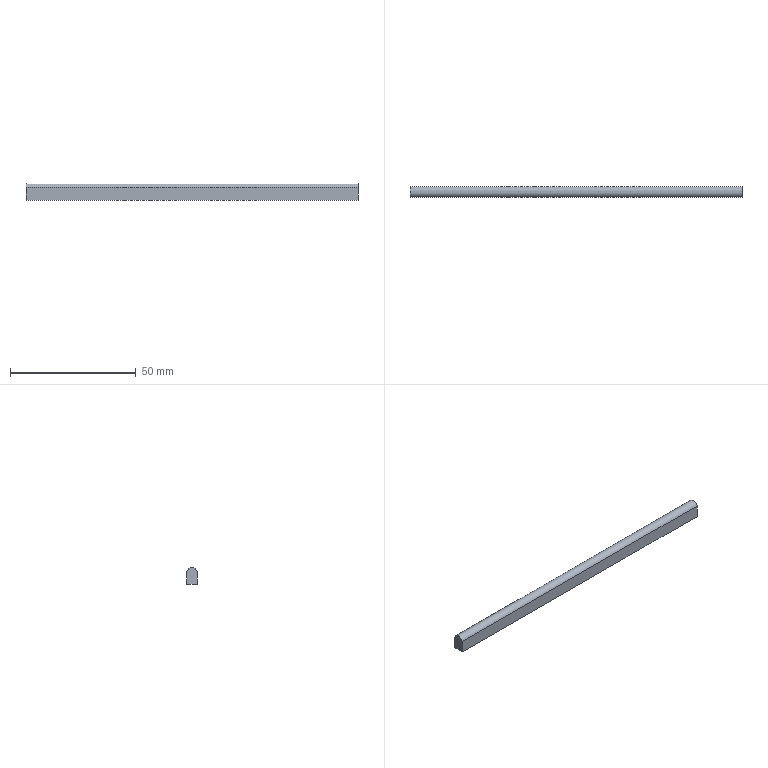CAM job | Mastercam | mm | 10 operations | part box 131.92 x 4.2 x 6.7
1. Facing | 10 - 10 平铣刀
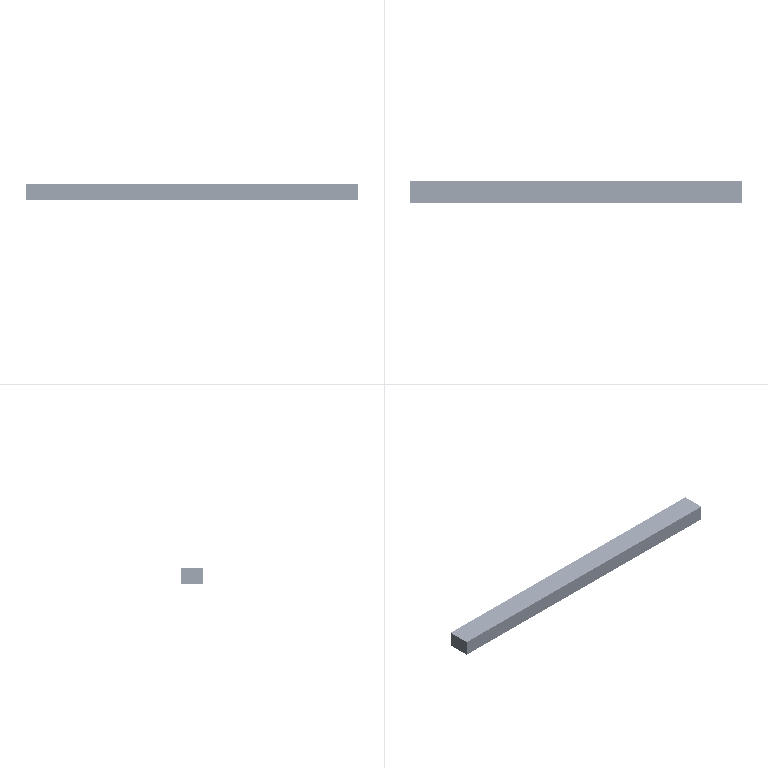2. 2D High Speed (2D Dynamic Mill) | 12 - 12 平铣刀
3. Contour (2D) | 10 - 10 平铣刀
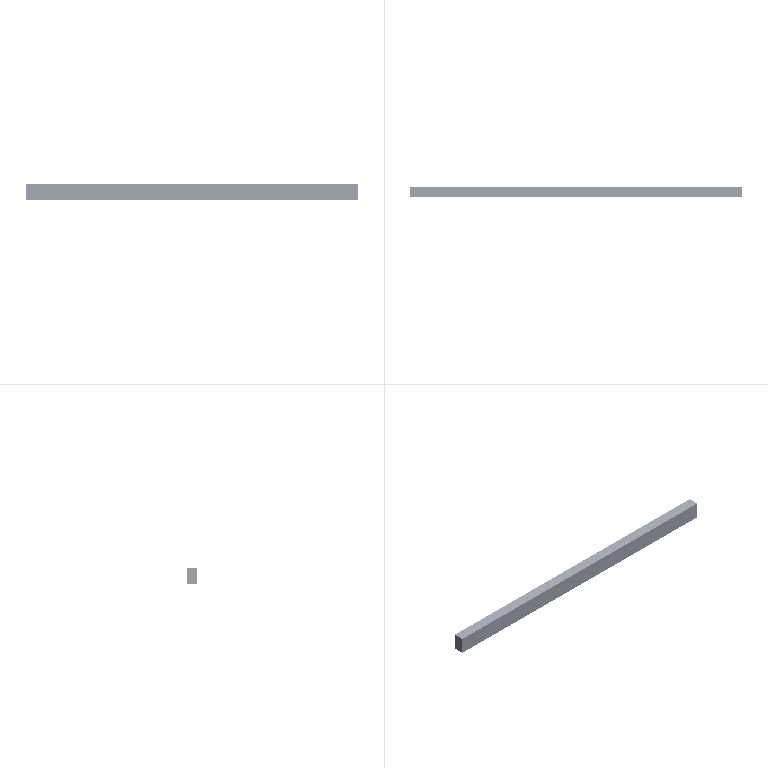4. Contour (2D chamfer) | 7 - 4 倒角刀
5. Facing | 12 - 12 平铣刀
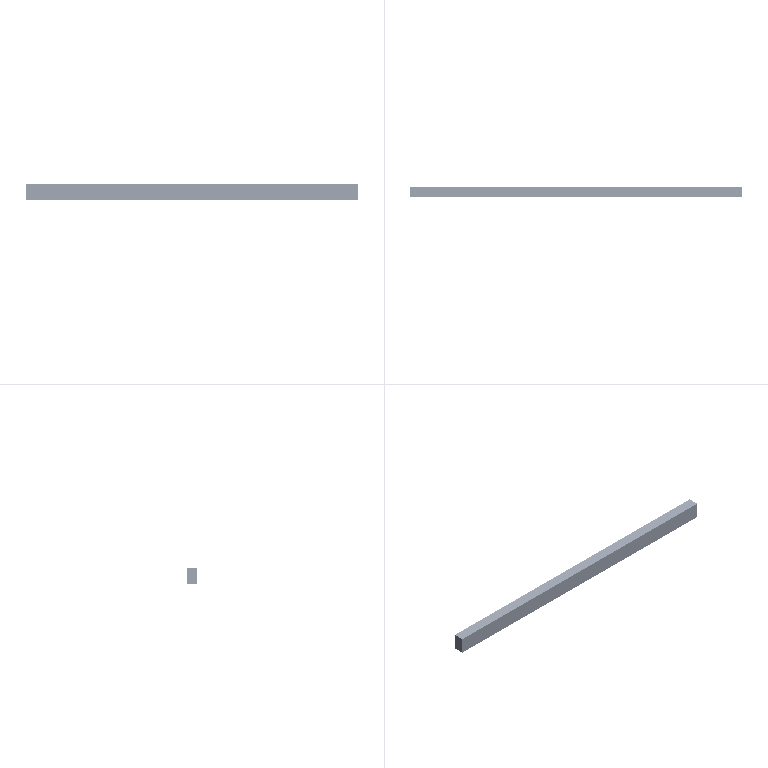6. Facing | 10 - 10 平铣刀
7. Surface Finish Flowline | 5 - 6 球刀/圆鼻铣刀
8. Facing | 10 - 10 平铣刀
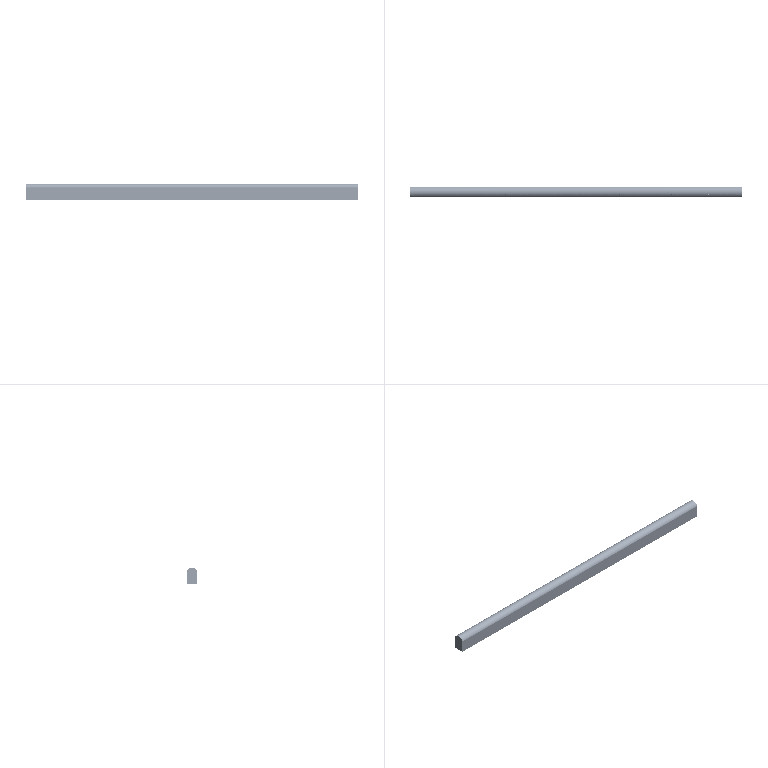9. Contour (2D chamfer) | 7 - 4 倒角刀
10. Contour (2D) | 9 - 8 平铣刀